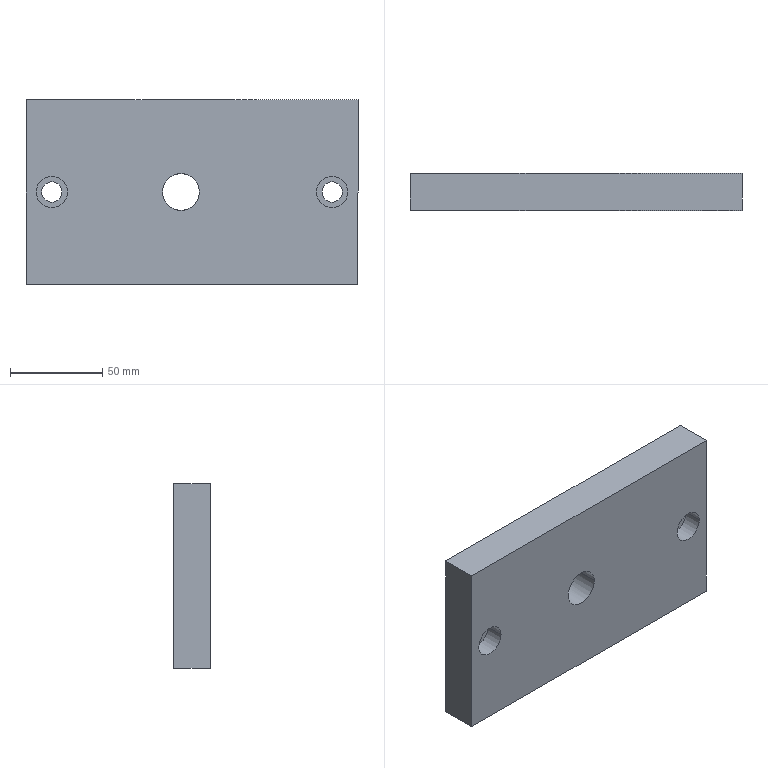Component | SolidWorks | SHYTJ-01-07-04PressurePlate-1 | 1 solid | 24 faces | box 180 x 20 x 100 mm | volume 345962 mm3 | cylinder 14 | plane 10 | commonest cylinder face diameters 20 x6 17 x4 11 x4
build123d program:
from build123d import *

# Parameters (mm, degrees)
SKETCH1_2_W             = 180
SKETCH1_2_H             = 100
BOSS_EXTRUDE1_DEPTH     = 20
SKETCH2_R               = 5
CUT_EXTRUDE1_2_DEPTH    = 207.882
SKETCH3_R               = 5.5
CUT_EXTRUDE2_DEPTH      = 207.882
SKETCH5_R               = 10
CUT_EXTRUDE3_DEPTH      = 3
SKETCH9_R               = 8.5
CUT_EXTRUDE4_DEPTH      = 10
M20X1_5_TAPPED_HOLE1_D  = 18.5
CUT_EXTRUDE1_DEPTH      = 207.882
CUT_EXTRUDE1_DEPTH_BACK = 207.882
SKETCH1_R               = 10


with BuildPart() as part:
    # Sketch1_2 → Boss-Extrude1 (new body)
    with BuildSketch(Plane.XY):
        with Locations((90, -50)):
            Rectangle(SKETCH1_2_W, SKETCH1_2_H)
    extrude(amount=BOSS_EXTRUDE1_DEPTH)

    # Sketch2 → Cut-Extrude1_2 (cut, through all)
    with BuildSketch(Plane.XY.offset(20)):
        with Locations((84, -50)):
            Circle(SKETCH2_R)
    extrude(amount=-CUT_EXTRUDE1_2_DEPTH, mode=Mode.SUBTRACT)

    # Sketch3 → Cut-Extrude2 (cut, through all)
    with BuildSketch(Plane.XY.offset(20)):
        with Locations((14, -50)):
            Circle(SKETCH3_R)
        with Locations((166, -50)):
            Circle(SKETCH3_R)
    extrude(amount=-CUT_EXTRUDE2_DEPTH, mode=Mode.SUBTRACT)

    # Sketch5 → Cut-Extrude3 (cut)
    with BuildSketch(Plane(origin=(0, 0, 0), x_dir=(-1, 0, 0), z_dir=(0, 0, -1))):
        with Locations((-14, -50)):
            Circle(SKETCH5_R)
        with Locations((-166, -50)):
            Circle(SKETCH5_R)
    extrude(amount=-CUT_EXTRUDE3_DEPTH, mode=Mode.SUBTRACT)

    # Sketch9 → Cut-Extrude4 (cut)
    with BuildSketch(Plane.XY.offset(20)):
        with Locations((14, -50)):
            Circle(SKETCH9_R)
        with Locations((166, -50)):
            Circle(SKETCH9_R)
    extrude(amount=-CUT_EXTRUDE4_DEPTH, mode=Mode.SUBTRACT)

    # M20x1.5 Tapped Hole1 (through all)
    with Locations(Plane.XY.offset(20)):
        with Locations((84, -50)):
            Hole(M20X1_5_TAPPED_HOLE1_D / 2)

    # Sketch1 → Cut-Extrude1 (cut, two sides: drawn at the far end of the back side and taken through both)
    with BuildSketch(Plane.XY.offset(-CUT_EXTRUDE1_DEPTH_BACK)):
        with Locations((84, -50)):
            Circle(SKETCH1_R)
    extrude(amount=CUT_EXTRUDE1_DEPTH + CUT_EXTRUDE1_DEPTH_BACK, mode=Mode.SUBTRACT)


solid = part.part

# Placed as in the assembly
solid = solid.moved(Location((-64.116, -45.361, 320), (90, 0, 0)))
STEP:
#1=COLOUR_RGB('',0.7922,0.8196,0.9333);
#2=FILL_AREA_STYLE_COLOUR('',#1);
#3=FILL_AREA_STYLE('',(#2));
#4=SURFACE_STYLE_FILL_AREA(#3);
#5=SURFACE_SIDE_STYLE('',(#4));
#6=SURFACE_STYLE_USAGE(.BOTH.,#5);
#7=PRESENTATION_STYLE_ASSIGNMENT((#6));
#8=CARTESIAN_POINT('',(0.3891,-1.786,10.63));
#9=VERTEX_POINT('',#8);
#10=CARTESIAN_POINT('',(1.177,-1.786,10.63));
#11=VERTEX_POINT('',#10);
#12=CARTESIAN_POINT('',(0.3891,-1.786,10.63));
#13=CARTESIAN_POINT('',(0.3891,-1.786,10.578));
#14=CARTESIAN_POINT('',(0.3991,-1.786,10.527));
#15=CARTESIAN_POINT('',(0.4391,-1.786,10.431));
#16=CARTESIAN_POINT('',(0.4675,-1.786,10.388));
#17=CARTESIAN_POINT('',(0.5414,-1.786,10.315));
#18=CARTESIAN_POINT('',(0.584,-1.786,10.286));
#19=CARTESIAN_POINT('',(0.6804,-1.786,10.246));
#20=CARTESIAN_POINT('',(0.7306,-1.786,10.236));
#21=CARTESIAN_POINT('',(0.835,-1.786,10.236));
#22=CARTESIAN_POINT('',(0.8853,-1.786,10.246));
#23=CARTESIAN_POINT('',(0.9817,-1.786,10.286));
#24=CARTESIAN_POINT('',(1.024,-1.786,10.315));
#25=CARTESIAN_POINT('',(1.098,-1.786,10.388));
#26=CARTESIAN_POINT('',(1.127,-1.786,10.431));
#27=CARTESIAN_POINT('',(1.167,-1.786,10.527));
#28=CARTESIAN_POINT('',(1.177,-1.786,10.578));
#29=CARTESIAN_POINT('',(1.177,-1.786,10.63));
#30=B_SPLINE_CURVE_WITH_KNOTS('',3,(#12,#13,#14,#15,#16,#17,#18,#19,#20,#21,#22,#23,#24,#25,#26,#27,#28,#29),.UNSPECIFIED.,.F.,.F.,(4,2,2,2,2,2,2,2,4),(0.5,0.5625,0.625,0.6875,0.75,0.8125,0.875,0.9375,1.),.UNSPECIFIED.);
#31=EDGE_CURVE('',#9,#11,#30,.T.);
#32=ORIENTED_EDGE('',*,*,#31,.F.);
#33=CARTESIAN_POINT('',(0.3891,-2.573,10.63));
#34=VERTEX_POINT('',#33);
#35=CARTESIAN_POINT('',(0.3891,-1.786,10.63));
#36=DIRECTION('',(-0.,-1.,-0.));
#37=VECTOR('',#36,39.37);
#38=LINE('',#35,#37);
#39=EDGE_CURVE('',#9,#34,#38,.T.);
#40=ORIENTED_EDGE('',*,*,#39,.T.);
#41=CARTESIAN_POINT('',(1.177,-2.573,10.63));
#42=VERTEX_POINT('',#41);
#43=CARTESIAN_POINT('',(0.7828,-2.573,10.63));
#44=DIRECTION('',(-0.,-1.,-0.));
#45=DIRECTION('',(1.,0.,0.));
#46=AXIS2_PLACEMENT_3D('',#43,#44,#45);
#47=CIRCLE('',#46,0.3937);
#48=EDGE_CURVE('',#34,#42,#47,.T.);
#49=ORIENTED_EDGE('',*,*,#48,.T.);
#50=CARTESIAN_POINT('',(1.177,-1.786,10.63));
#51=DIRECTION('',(-0.,-1.,-0.));
#52=VECTOR('',#51,39.37);
#53=LINE('',#50,#52);
#54=EDGE_CURVE('',#11,#42,#53,.T.);
#55=ORIENTED_EDGE('',*,*,#54,.F.);
#56=EDGE_LOOP('',(#32,#40,#49,#55));
#57=FACE_OUTER_BOUND('',#56,.T.);
#58=CARTESIAN_POINT('',(0.7828,-1.786,10.63));
#59=DIRECTION('',(-0.,-1.,-0.));
#60=DIRECTION('',(1.,0.,0.));
#61=AXIS2_PLACEMENT_3D('',#58,#59,#60);
#62=CYLINDRICAL_SURFACE('',#61,0.3937);
#63=ADVANCED_FACE('',(#57),#62,.F.);
#64=CARTESIAN_POINT('',(3.677,-2.18,10.63));
#65=VERTEX_POINT('',#64);
#66=CARTESIAN_POINT('',(4.346,-2.18,10.63));
#67=VERTEX_POINT('',#66);
#68=CARTESIAN_POINT('',(4.011,-2.18,10.63));
#69=DIRECTION('',(-0.,-1.,-0.));
#70=DIRECTION('',(1.,0.,0.));
#71=AXIS2_PLACEMENT_3D('',#68,#69,#70);
#72=CIRCLE('',#71,0.3346);
#73=EDGE_CURVE('',#65,#67,#72,.T.);
#74=ORIENTED_EDGE('',*,*,#73,.F.);
#75=CARTESIAN_POINT('',(3.677,-2.573,10.63));
#76=VERTEX_POINT('',#75);
#77=CARTESIAN_POINT('',(3.677,-2.18,10.63));
#78=DIRECTION('',(-0.,-1.,-0.));
#79=VECTOR('',#78,39.37);
#80=LINE('',#77,#79);
#81=EDGE_CURVE('',#65,#76,#80,.T.);
#82=ORIENTED_EDGE('',*,*,#81,.T.);
#83=CARTESIAN_POINT('',(4.346,-2.573,10.63));
#84=VERTEX_POINT('',#83);
#85=CARTESIAN_POINT('',(4.011,-2.573,10.63));
#86=DIRECTION('',(-0.,-1.,-0.));
#87=DIRECTION('',(1.,0.,0.));
#88=AXIS2_PLACEMENT_3D('',#85,#86,#87);
#89=CIRCLE('',#88,0.3346);
#90=EDGE_CURVE('',#76,#84,#89,.T.);
#91=ORIENTED_EDGE('',*,*,#90,.T.);
#92=CARTESIAN_POINT('',(4.346,-2.18,10.63));
#93=DIRECTION('',(-0.,-1.,-0.));
#94=VECTOR('',#93,39.37);
#95=LINE('',#92,#94);
#96=EDGE_CURVE('',#67,#84,#95,.T.);
#97=ORIENTED_EDGE('',*,*,#96,.F.);
#98=EDGE_LOOP('',(#74,#82,#91,#97));
#99=FACE_OUTER_BOUND('',#98,.T.);
#100=CARTESIAN_POINT('',(4.011,-2.18,10.63));
#101=DIRECTION('',(-0.,-1.,-0.));
#102=DIRECTION('',(1.,0.,0.));
#103=AXIS2_PLACEMENT_3D('',#100,#101,#102);
#104=CYLINDRICAL_SURFACE('',#103,0.3346);
#105=ADVANCED_FACE('',(#99),#104,.F.);
#106=CARTESIAN_POINT('',(-2.308,-2.18,10.63));
#107=VERTEX_POINT('',#106);
#108=CARTESIAN_POINT('',(-1.638,-2.18,10.63));
#109=VERTEX_POINT('',#108);
#110=CARTESIAN_POINT('',(-1.973,-2.18,10.63));
#111=DIRECTION('',(-0.,-1.,-0.));
#112=DIRECTION('',(1.,0.,0.));
#113=AXIS2_PLACEMENT_3D('',#110,#111,#112);
#114=CIRCLE('',#113,0.3346);
#115=EDGE_CURVE('',#107,#109,#114,.T.);
#116=ORIENTED_EDGE('',*,*,#115,.F.);
#117=CARTESIAN_POINT('',(-2.308,-2.573,10.63));
#118=VERTEX_POINT('',#117);
#119=CARTESIAN_POINT('',(-2.308,-2.18,10.63));
#120=DIRECTION('',(-0.,-1.,-0.));
#121=VECTOR('',#120,39.37);
#122=LINE('',#119,#121);
#123=EDGE_CURVE('',#107,#118,#122,.T.);
#124=ORIENTED_EDGE('',*,*,#123,.T.);
#125=CARTESIAN_POINT('',(-1.638,-2.573,10.63));
#126=VERTEX_POINT('',#125);
#127=CARTESIAN_POINT('',(-1.973,-2.573,10.63));
#128=DIRECTION('',(-0.,-1.,-0.));
#129=DIRECTION('',(1.,0.,0.));
#130=AXIS2_PLACEMENT_3D('',#127,#128,#129);
#131=CIRCLE('',#130,0.3346);
#132=EDGE_CURVE('',#118,#126,#131,.T.);
#133=ORIENTED_EDGE('',*,*,#132,.T.);
#134=CARTESIAN_POINT('',(-1.638,-2.18,10.63));
#135=DIRECTION('',(-0.,-1.,-0.));
#136=VECTOR('',#135,39.37);
#137=LINE('',#134,#136);
#138=EDGE_CURVE('',#109,#126,#137,.T.);
#139=ORIENTED_EDGE('',*,*,#138,.F.);
#140=EDGE_LOOP('',(#116,#124,#133,#139));
#141=FACE_OUTER_BOUND('',#140,.T.);
#142=CARTESIAN_POINT('',(-1.973,-2.18,10.63));
#143=DIRECTION('',(-0.,-1.,-0.));
#144=DIRECTION('',(1.,0.,0.));
#145=AXIS2_PLACEMENT_3D('',#142,#143,#144);
#146=CYLINDRICAL_SURFACE('',#145,0.3346);
#147=ADVANCED_FACE('',(#141),#146,.F.);
#148=CARTESIAN_POINT('',(4.405,-1.904,10.63));
#149=VERTEX_POINT('',#148);
#150=CARTESIAN_POINT('',(3.617,-1.904,10.63));
#151=VERTEX_POINT('',#150);
#152=CARTESIAN_POINT('',(4.011,-1.904,10.63));
#153=DIRECTION('',(0.,1.,0.));
#154=DIRECTION('',(-1.,0.,0.));
#155=AXIS2_PLACEMENT_3D('',#152,#153,#154);
#156=CIRCLE('',#155,0.3937);
#157=EDGE_CURVE('',#149,#151,#156,.T.);
#158=ORIENTED_EDGE('',*,*,#157,.F.);
#159=CARTESIAN_POINT('',(4.405,-1.786,10.63));
#160=VERTEX_POINT('',#159);
#161=CARTESIAN_POINT('',(4.405,-1.904,10.63));
#162=DIRECTION('',(0.,1.,0.));
#163=VECTOR('',#162,39.37);
#164=LINE('',#161,#163);
#165=EDGE_CURVE('',#149,#160,#164,.T.);
#166=ORIENTED_EDGE('',*,*,#165,.T.);
#167=CARTESIAN_POINT('',(3.617,-1.786,10.63));
#168=VERTEX_POINT('',#167);
#169=CARTESIAN_POINT('',(4.011,-1.786,10.63));
#170=DIRECTION('',(0.,1.,0.));
#171=DIRECTION('',(-1.,0.,0.));
#172=AXIS2_PLACEMENT_3D('',#169,#170,#171);
#173=CIRCLE('',#172,0.3937);
#174=EDGE_CURVE('',#160,#168,#173,.T.);
#175=ORIENTED_EDGE('',*,*,#174,.T.);
#176=CARTESIAN_POINT('',(3.617,-1.904,10.63));
#177=DIRECTION('',(0.,1.,0.));
#178=VECTOR('',#177,39.37);
#179=LINE('',#176,#178);
#180=EDGE_CURVE('',#151,#168,#179,.T.);
#181=ORIENTED_EDGE('',*,*,#180,.F.);
#182=EDGE_LOOP('',(#158,#166,#175,#181));
#183=FACE_OUTER_BOUND('',#182,.T.);
#184=CARTESIAN_POINT('',(4.011,-1.904,10.63));
#185=DIRECTION('',(0.,1.,0.));
#186=DIRECTION('',(-1.,0.,0.));
#187=AXIS2_PLACEMENT_3D('',#184,#185,#186);
#188=CYLINDRICAL_SURFACE('',#187,0.3937);
#189=ADVANCED_FACE('',(#183),#188,.F.);
#190=CARTESIAN_POINT('',(-1.579,-1.904,10.63));
#191=VERTEX_POINT('',#190);
#192=CARTESIAN_POINT('',(-2.367,-1.904,10.63));
#193=VERTEX_POINT('',#192);
#194=CARTESIAN_POINT('',(-1.973,-1.904,10.63));
#195=DIRECTION('',(0.,1.,0.));
#196=DIRECTION('',(-1.,0.,0.));
#197=AXIS2_PLACEMENT_3D('',#194,#195,#196);
#198=CIRCLE('',#197,0.3937);
#199=EDGE_CURVE('',#191,#193,#198,.T.);
#200=ORIENTED_EDGE('',*,*,#199,.F.);
#201=CARTESIAN_POINT('',(-1.579,-1.786,10.63));
#202=VERTEX_POINT('',#201);
#203=CARTESIAN_POINT('',(-1.579,-1.904,10.63));
#204=DIRECTION('',(0.,1.,0.));
#205=VECTOR('',#204,39.37);
#206=LINE('',#203,#205);
#207=EDGE_CURVE('',#191,#202,#206,.T.);
#208=ORIENTED_EDGE('',*,*,#207,.T.);
#209=CARTESIAN_POINT('',(-2.367,-1.786,10.63));
#210=VERTEX_POINT('',#209);
#211=CARTESIAN_POINT('',(-1.973,-1.786,10.63));
#212=DIRECTION('',(0.,1.,0.));
#213=DIRECTION('',(-1.,0.,0.));
#214=AXIS2_PLACEMENT_3D('',#211,#212,#213);
#215=CIRCLE('',#214,0.3937);
#216=EDGE_CURVE('',#202,#210,#215,.T.);
#217=ORIENTED_EDGE('',*,*,#216,.T.);
#218=CARTESIAN_POINT('',(-2.367,-1.904,10.63));
#219=DIRECTION('',(0.,1.,0.));
#220=VECTOR('',#219,39.37);
#221=LINE('',#218,#220);
#222=EDGE_CURVE('',#193,#210,#221,.T.);
#223=ORIENTED_EDGE('',*,*,#222,.F.);
#224=EDGE_LOOP('',(#200,#208,#217,#223));
#225=FACE_OUTER_BOUND('',#224,.T.);
#226=CARTESIAN_POINT('',(-1.973,-1.904,10.63));
#227=DIRECTION('',(0.,1.,0.));
#228=DIRECTION('',(-1.,0.,0.));
#229=AXIS2_PLACEMENT_3D('',#226,#227,#228);
#230=CYLINDRICAL_SURFACE('',#229,0.3937);
#231=ADVANCED_FACE('',(#225),#230,.F.);
#232=CARTESIAN_POINT('',(-2.19,-1.904,10.63));
#233=VERTEX_POINT('',#232);
#234=CARTESIAN_POINT('',(-1.757,-1.904,10.63));
#235=VERTEX_POINT('',#234);
#236=CARTESIAN_POINT('',(-1.973,-1.904,10.63));
#237=DIRECTION('',(-0.,-1.,-0.));
#238=DIRECTION('',(-1.,0.,0.));
#239=AXIS2_PLACEMENT_3D('',#236,#237,#238);
#240=CIRCLE('',#239,0.2165);
#241=EDGE_CURVE('',#233,#235,#240,.T.);
#242=ORIENTED_EDGE('',*,*,#241,.F.);
#243=CARTESIAN_POINT('',(-2.19,-2.18,10.63));
#244=VERTEX_POINT('',#243);
#245=CARTESIAN_POINT('',(-2.19,-1.786,10.63));
#246=DIRECTION('',(-0.,-1.,-0.));
#247=VECTOR('',#246,39.37);
#248=LINE('',#245,#247);
#249=EDGE_CURVE('',#233,#244,#248,.T.);
#250=ORIENTED_EDGE('',*,*,#249,.T.);
#251=CARTESIAN_POINT('',(-1.757,-2.18,10.63));
#252=VERTEX_POINT('',#251);
#253=CARTESIAN_POINT('',(-1.973,-2.18,10.63));
#254=DIRECTION('',(0.,1.,0.));
#255=DIRECTION('',(1.,0.,0.));
#256=AXIS2_PLACEMENT_3D('',#253,#254,#255);
#257=CIRCLE('',#256,0.2165);
#258=EDGE_CURVE('',#252,#244,#257,.T.);
#259=ORIENTED_EDGE('',*,*,#258,.F.);
#260=CARTESIAN_POINT('',(-1.757,-1.786,10.63));
#261=DIRECTION('',(-0.,-1.,-0.));
#262=VECTOR('',#261,39.37);
#263=LINE('',#260,#262);
#264=EDGE_CURVE('',#235,#252,#263,.T.);
#265=ORIENTED_EDGE('',*,*,#264,.F.);
#266=EDGE_LOOP('',(#242,#250,#259,#265));
#267=FACE_OUTER_BOUND('',#266,.T.);
#268=CARTESIAN_POINT('',(-1.973,-1.786,10.63));
#269=DIRECTION('',(-0.,-1.,-0.));
#270=DIRECTION('',(1.,0.,0.));
#271=AXIS2_PLACEMENT_3D('',#268,#269,#270);
#272=CYLINDRICAL_SURFACE('',#271,0.2165);
#273=ADVANCED_FACE('',(#267),#272,.F.);
#274=CARTESIAN_POINT('',(3.795,-1.904,10.63));
#275=VERTEX_POINT('',#274);
#276=CARTESIAN_POINT('',(4.228,-1.904,10.63));
#277=VERTEX_POINT('',#276);
#278=CARTESIAN_POINT('',(4.011,-1.904,10.63));
#279=DIRECTION('',(-0.,-1.,-0.));
#280=DIRECTION('',(-1.,0.,0.));
#281=AXIS2_PLACEMENT_3D('',#278,#279,#280);
#282=CIRCLE('',#281,0.2165);
#283=EDGE_CURVE('',#275,#277,#282,.T.);
#284=ORIENTED_EDGE('',*,*,#283,.F.);
#285=CARTESIAN_POINT('',(3.795,-2.18,10.63));
#286=VERTEX_POINT('',#285);
#287=CARTESIAN_POINT('',(3.795,-1.786,10.63));
#288=DIRECTION('',(-0.,-1.,-0.));
#289=VECTOR('',#288,39.37);
#290=LINE('',#287,#289);
#291=EDGE_CURVE('',#275,#286,#290,.T.);
#292=ORIENTED_EDGE('',*,*,#291,.T.);
#293=CARTESIAN_POINT('',(4.228,-2.18,10.63));
#294=VERTEX_POINT('',#293);
#295=CARTESIAN_POINT('',(4.011,-2.18,10.63));
#296=DIRECTION('',(0.,1.,0.));
#297=DIRECTION('',(1.,0.,0.));
#298=AXIS2_PLACEMENT_3D('',#295,#296,#297);
#299=CIRCLE('',#298,0.2165);
#300=EDGE_CURVE('',#294,#286,#299,.T.);
#301=ORIENTED_EDGE('',*,*,#300,.F.);
#302=CARTESIAN_POINT('',(4.228,-1.786,10.63));
#303=DIRECTION('',(-0.,-1.,-0.));
#304=VECTOR('',#303,39.37);
#305=LINE('',#302,#304);
#306=EDGE_CURVE('',#277,#294,#305,.T.);
#307=ORIENTED_EDGE('',*,*,#306,.F.);
#308=EDGE_LOOP('',(#284,#292,#301,#307));
#309=FACE_OUTER_BOUND('',#308,.T.);
#310=CARTESIAN_POINT('',(4.011,-1.786,10.63));
#311=DIRECTION('',(-0.,-1.,-0.));
#312=DIRECTION('',(1.,0.,0.));
#313=AXIS2_PLACEMENT_3D('',#310,#311,#312);
#314=CYLINDRICAL_SURFACE('',#313,0.2165);
#315=ADVANCED_FACE('',(#309),#314,.F.);
#316=ORIENTED_EDGE('',*,*,#291,.F.);
#317=CARTESIAN_POINT('',(4.011,-1.904,10.63));
#318=DIRECTION('',(-0.,-1.,-0.));
#319=DIRECTION('',(-1.,0.,0.));
#320=AXIS2_PLACEMENT_3D('',#317,#318,#319);
#321=CIRCLE('',#320,0.2165);
#322=EDGE_CURVE('',#277,#275,#321,.T.);
#323=ORIENTED_EDGE('',*,*,#322,.F.);
#324=ORIENTED_EDGE('',*,*,#306,.T.);
#325=CARTESIAN_POINT('',(4.011,-2.18,10.63));
#326=DIRECTION('',(0.,1.,0.));
#327=DIRECTION('',(1.,0.,0.));
#328=AXIS2_PLACEMENT_3D('',#325,#326,#327);
#329=CIRCLE('',#328,0.2165);
#330=EDGE_CURVE('',#286,#294,#329,.T.);
#331=ORIENTED_EDGE('',*,*,#330,.F.);
#332=EDGE_LOOP('',(#316,#323,#324,#331));
#333=FACE_OUTER_BOUND('',#332,.T.);
#334=CARTESIAN_POINT('',(4.011,-1.786,10.63));
#335=DIRECTION('',(-0.,-1.,-0.));
#336=DIRECTION('',(1.,0.,0.));
#337=AXIS2_PLACEMENT_3D('',#334,#335,#336);
#338=CYLINDRICAL_SURFACE('',#337,0.2165);
#339=ADVANCED_FACE('',(#333),#338,.F.);
#340=ORIENTED_EDGE('',*,*,#249,.F.);
#341=CARTESIAN_POINT('',(-1.973,-1.904,10.63));
#342=DIRECTION('',(-0.,-1.,-0.));
#343=DIRECTION('',(-1.,0.,0.));
#344=AXIS2_PLACEMENT_3D('',#341,#342,#343);
#345=CIRCLE('',#344,0.2165);
#346=EDGE_CURVE('',#235,#233,#345,.T.);
#347=ORIENTED_EDGE('',*,*,#346,.F.);
#348=ORIENTED_EDGE('',*,*,#264,.T.);
#349=CARTESIAN_POINT('',(-1.973,-2.18,10.63));
#350=DIRECTION('',(0.,1.,0.));
#351=DIRECTION('',(1.,0.,0.));
#352=AXIS2_PLACEMENT_3D('',#349,#350,#351);
#353=CIRCLE('',#352,0.2165);
#354=EDGE_CURVE('',#244,#252,#353,.T.);
#355=ORIENTED_EDGE('',*,*,#354,.F.);
#356=EDGE_LOOP('',(#340,#347,#348,#355));
#357=FACE_OUTER_BOUND('',#356,.T.);
#358=CARTESIAN_POINT('',(-1.973,-1.786,10.63));
#359=DIRECTION('',(-0.,-1.,-0.));
#360=DIRECTION('',(1.,0.,0.));
#361=AXIS2_PLACEMENT_3D('',#358,#359,#360);
#362=CYLINDRICAL_SURFACE('',#361,0.2165);
#363=ADVANCED_FACE('',(#357),#362,.F.);
#364=CARTESIAN_POINT('',(-2.524,-1.786,12.598));
#365=VERTEX_POINT('',#364);
#366=CARTESIAN_POINT('',(-2.524,-1.786,8.661));
#367=VERTEX_POINT('',#366);
#368=CARTESIAN_POINT('',(-2.524,-1.786,12.598));
#369=DIRECTION('',(-0.,0.,-1.));
#370=VECTOR('',#369,39.37);
#371=LINE('',#368,#370);
#372=EDGE_CURVE('',#365,#367,#371,.T.);
#373=ORIENTED_EDGE('',*,*,#372,.T.);
#374=CARTESIAN_POINT('',(-2.524,-2.573,8.661));
#375=VERTEX_POINT('',#374);
#376=CARTESIAN_POINT('',(-2.524,-2.573,8.661));
#377=DIRECTION('',(0.,1.,0.));
#378=VECTOR('',#377,39.37);
#379=LINE('',#376,#378);
#380=EDGE_CURVE('',#375,#367,#379,.T.);
#381=ORIENTED_EDGE('',*,*,#380,.F.);
#382=CARTESIAN_POINT('',(-2.524,-2.573,12.598));
#383=VERTEX_POINT('',#382);
#384=CARTESIAN_POINT('',(-2.524,-2.573,12.598));
#385=DIRECTION('',(-0.,0.,-1.));
#386=VECTOR('',#385,39.37);
#387=LINE('',#384,#386);
#388=EDGE_CURVE('',#383,#375,#387,.T.);
#389=ORIENTED_EDGE('',*,*,#388,.F.);
#390=CARTESIAN_POINT('',(-2.524,-2.573,12.598));
#391=DIRECTION('',(0.,1.,0.));
#392=VECTOR('',#391,39.37);
#393=LINE('',#390,#392);
#394=EDGE_CURVE('',#383,#365,#393,.T.);
#395=ORIENTED_EDGE('',*,*,#394,.T.);
#396=EDGE_LOOP('',(#373,#381,#389,#395));
#397=FACE_OUTER_BOUND('',#396,.T.);
#398=CARTESIAN_POINT('',(-2.524,-2.573,12.598));
#399=DIRECTION('',(1.,-0.,-0.));
#400=DIRECTION('',(0.,-0.,1.));
#401=AXIS2_PLACEMENT_3D('',#398,#399,#400);
#402=PLANE('',#401);
#403=ADVANCED_FACE('',(#397),#402,.F.);
#404=CARTESIAN_POINT('',(4.562,-1.786,8.661));
#405=VERTEX_POINT('',#404);
#406=CARTESIAN_POINT('',(-2.524,-1.786,8.661));
#407=DIRECTION('',(1.,-0.,-0.));
#408=VECTOR('',#407,39.37);
#409=LINE('',#406,#408);
#410=EDGE_CURVE('',#367,#405,#409,.T.);
#411=ORIENTED_EDGE('',*,*,#410,.T.);
#412=CARTESIAN_POINT('',(4.562,-2.573,8.661));
#413=VERTEX_POINT('',#412);
#414=CARTESIAN_POINT('',(4.562,-2.573,8.661));
#415=DIRECTION('',(0.,1.,0.));
#416=VECTOR('',#415,39.37);
#417=LINE('',#414,#416);
#418=EDGE_CURVE('',#413,#405,#417,.T.);
#419=ORIENTED_EDGE('',*,*,#418,.F.);
#420=CARTESIAN_POINT('',(-2.524,-2.573,8.661));
#421=DIRECTION('',(1.,-0.,-0.));
#422=VECTOR('',#421,39.37);
#423=LINE('',#420,#422);
#424=EDGE_CURVE('',#375,#413,#423,.T.);
#425=ORIENTED_EDGE('',*,*,#424,.F.);
#426=ORIENTED_EDGE('',*,*,#380,.T.);
#427=EDGE_LOOP('',(#411,#419,#425,#426));
#428=FACE_OUTER_BOUND('',#427,.T.);
#429=CARTESIAN_POINT('',(-2.524,-2.573,8.661));
#430=DIRECTION('',(0.,-0.,1.));
#431=DIRECTION('',(-0.,-1.,-0.));
#432=AXIS2_PLACEMENT_3D('',#429,#430,#431);
#433=PLANE('',#432);
#434=ADVANCED_FACE('',(#428),#433,.F.);
#435=CARTESIAN_POINT('',(4.562,-1.786,12.598));
#436=VERTEX_POINT('',#435);
#437=CARTESIAN_POINT('',(4.562,-1.786,12.598));
#438=DIRECTION('',(0.,-0.,1.));
#439=VECTOR('',#438,39.37);
#440=LINE('',#437,#439);
#441=EDGE_CURVE('',#405,#436,#440,.T.);
#442=ORIENTED_EDGE('',*,*,#441,.T.);
#443=CARTESIAN_POINT('',(4.562,-2.573,12.598));
#444=VERTEX_POINT('',#443);
#445=CARTESIAN_POINT('',(4.562,-2.573,12.598));
#446=DIRECTION('',(0.,1.,0.));
#447=VECTOR('',#446,39.37);
#448=LINE('',#445,#447);
#449=EDGE_CURVE('',#444,#436,#448,.T.);
#450=ORIENTED_EDGE('',*,*,#449,.F.);
#451=CARTESIAN_POINT('',(4.562,-2.573,12.598));
#452=DIRECTION('',(0.,-0.,1.));
#453=VECTOR('',#452,39.37);
#454=LINE('',#451,#453);
#455=EDGE_CURVE('',#413,#444,#454,.T.);
#456=ORIENTED_EDGE('',*,*,#455,.F.);
#457=ORIENTED_EDGE('',*,*,#418,.T.);
#458=EDGE_LOOP('',(#442,#450,#456,#457));
#459=FACE_OUTER_BOUND('',#458,.T.);
#460=CARTESIAN_POINT('',(4.562,-2.573,12.598));
#461=DIRECTION('',(-1.,0.,0.));
#462=DIRECTION('',(-0.,-1.,-0.));
#463=AXIS2_PLACEMENT_3D('',#460,#461,#462);
#464=PLANE('',#463);
#465=ADVANCED_FACE('',(#459),#464,.F.);
#466=CARTESIAN_POINT('',(-2.524,-1.786,12.598));
#467=DIRECTION('',(-1.,0.,0.));
#468=VECTOR('',#467,39.37);
#469=LINE('',#466,#468);
#470=EDGE_CURVE('',#436,#365,#469,.T.);
#471=ORIENTED_EDGE('',*,*,#470,.T.);
#472=ORIENTED_EDGE('',*,*,#394,.F.);
#473=CARTESIAN_POINT('',(-2.524,-2.573,12.598));
#474=DIRECTION('',(-1.,0.,0.));
#475=VECTOR('',#474,39.37);
#476=LINE('',#473,#475);
#477=EDGE_CURVE('',#444,#383,#476,.T.);
#478=ORIENTED_EDGE('',*,*,#477,.F.);
#479=ORIENTED_EDGE('',*,*,#449,.T.);
#480=EDGE_LOOP('',(#471,#472,#478,#479));
#481=FACE_OUTER_BOUND('',#480,.T.);
#482=CARTESIAN_POINT('',(-2.524,-2.573,12.598));
#483=DIRECTION('',(-0.,0.,-1.));
#484=DIRECTION('',(0.,1.,0.));
#485=AXIS2_PLACEMENT_3D('',#482,#483,#484);
#486=PLANE('',#485);
#487=ADVANCED_FACE('',(#481),#486,.F.);
#488=CARTESIAN_POINT('',(0.7828,-2.573,10.63));
#489=DIRECTION('',(-0.,-1.,-0.));
#490=DIRECTION('',(1.,0.,0.));
#491=AXIS2_PLACEMENT_3D('',#488,#489,#490);
#492=CIRCLE('',#491,0.3937);
#493=EDGE_CURVE('',#42,#34,#492,.T.);
#494=ORIENTED_EDGE('',*,*,#493,.F.);
#495=ORIENTED_EDGE('',*,*,#48,.F.);
#496=EDGE_LOOP('',(#494,#495));
#497=FACE_BOUND('',#496,.T.);
#498=CARTESIAN_POINT('',(4.011,-2.573,10.63));
#499=DIRECTION('',(-0.,-1.,-0.));
#500=DIRECTION('',(1.,0.,0.));
#501=AXIS2_PLACEMENT_3D('',#498,#499,#500);
#502=CIRCLE('',#501,0.3346);
#503=EDGE_CURVE('',#84,#76,#502,.T.);
#504=ORIENTED_EDGE('',*,*,#503,.F.);
#505=ORIENTED_EDGE('',*,*,#90,.F.);
#506=EDGE_LOOP('',(#504,#505));
#507=FACE_BOUND('',#506,.T.);
#508=CARTESIAN_POINT('',(-1.973,-2.573,10.63));
#509=DIRECTION('',(-0.,-1.,-0.));
#510=DIRECTION('',(1.,0.,0.));
#511=AXIS2_PLACEMENT_3D('',#508,#509,#510);
#512=CIRCLE('',#511,0.3346);
#513=EDGE_CURVE('',#126,#118,#512,.T.);
#514=ORIENTED_EDGE('',*,*,#513,.F.);
#515=ORIENTED_EDGE('',*,*,#132,.F.);
#516=EDGE_LOOP('',(#514,#515));
#517=FACE_BOUND('',#516,.T.);
#518=ORIENTED_EDGE('',*,*,#388,.T.);
#519=ORIENTED_EDGE('',*,*,#424,.T.);
#520=ORIENTED_EDGE('',*,*,#455,.T.);
#521=ORIENTED_EDGE('',*,*,#477,.T.);
#522=EDGE_LOOP('',(#518,#519,#520,#521));
#523=FACE_OUTER_BOUND('',#522,.T.);
#524=CARTESIAN_POINT('',(-2.524,-2.573,12.598));
#525=DIRECTION('',(-0.,-1.,-0.));
#526=DIRECTION('',(1.,-0.,-0.));
#527=AXIS2_PLACEMENT_3D('',#524,#525,#526);
#528=PLANE('',#527);
#529=ADVANCED_FACE('',(#497,#507,#517,#523),#528,.T.);
#530=CARTESIAN_POINT('',(1.177,-1.786,10.63));
#531=CARTESIAN_POINT('',(1.177,-1.786,10.682));
#532=CARTESIAN_POINT('',(1.167,-1.786,10.732));
#533=CARTESIAN_POINT('',(1.127,-1.786,10.829));
#534=CARTESIAN_POINT('',(1.098,-1.786,10.871));
#535=CARTESIAN_POINT('',(1.024,-1.786,10.945));
#536=CARTESIAN_POINT('',(0.9817,-1.786,10.974));
#537=CARTESIAN_POINT('',(0.8853,-1.786,11.014));
#538=CARTESIAN_POINT('',(0.835,-1.786,11.024));
#539=CARTESIAN_POINT('',(0.7306,-1.786,11.024));
#540=CARTESIAN_POINT('',(0.6804,-1.786,11.014));
#541=CARTESIAN_POINT('',(0.584,-1.786,10.974));
#542=CARTESIAN_POINT('',(0.5414,-1.786,10.945));
#543=CARTESIAN_POINT('',(0.4675,-1.786,10.871));
#544=CARTESIAN_POINT('',(0.4391,-1.786,10.829));
#545=CARTESIAN_POINT('',(0.3991,-1.786,10.732));
#546=CARTESIAN_POINT('',(0.3891,-1.786,10.682));
#547=CARTESIAN_POINT('',(0.3891,-1.786,10.63));
#548=B_SPLINE_CURVE_WITH_KNOTS('',3,(#530,#531,#532,#533,#534,#535,#536,#537,#538,#539,#540,#541,#542,#543,#544,#545,#546,#547),.UNSPECIFIED.,.F.,.F.,(4,2,2,2,2,2,2,2,4),(0.,0.0625,0.125,0.1875,0.25,0.3125,0.375,0.4375,0.5),.UNSPECIFIED.);
#549=EDGE_CURVE('',#11,#9,#548,.T.);
#550=ORIENTED_EDGE('',*,*,#549,.T.);
#551=ORIENTED_EDGE('',*,*,#31,.T.);
#552=EDGE_LOOP('',(#550,#551));
#553=FACE_BOUND('',#552,.T.);
#554=CARTESIAN_POINT('',(4.011,-1.786,10.63));
#555=DIRECTION('',(0.,1.,0.));
#556=DIRECTION('',(-1.,0.,0.));
#557=AXIS2_PLACEMENT_3D('',#554,#555,#556);
#558=CIRCLE('',#557,0.3937);
#559=EDGE_CURVE('',#168,#160,#558,.T.);
#560=ORIENTED_EDGE('',*,*,#559,.F.);
#561=ORIENTED_EDGE('',*,*,#174,.F.);
#562=EDGE_LOOP('',(#560,#561));
#563=FACE_BOUND('',#562,.T.);
#564=CARTESIAN_POINT('',(-1.973,-1.786,10.63));
#565=DIRECTION('',(0.,1.,0.));
#566=DIRECTION('',(-1.,0.,0.));
#567=AXIS2_PLACEMENT_3D('',#564,#565,#566);
#568=CIRCLE('',#567,0.3937);
#569=EDGE_CURVE('',#210,#202,#568,.T.);
#570=ORIENTED_EDGE('',*,*,#569,.F.);
#571=ORIENTED_EDGE('',*,*,#216,.F.);
#572=EDGE_LOOP('',(#570,#571));
#573=FACE_BOUND('',#572,.T.);
#574=ORIENTED_EDGE('',*,*,#372,.F.);
#575=ORIENTED_EDGE('',*,*,#470,.F.);
#576=ORIENTED_EDGE('',*,*,#441,.F.);
#577=ORIENTED_EDGE('',*,*,#410,.F.);
#578=EDGE_LOOP('',(#574,#575,#576,#577));
#579=FACE_OUTER_BOUND('',#578,.T.);
#580=CARTESIAN_POINT('',(-2.524,-1.786,12.598));
#581=DIRECTION('',(-0.,-1.,-0.));
#582=DIRECTION('',(1.,-0.,-0.));
#583=AXIS2_PLACEMENT_3D('',#580,#581,#582);
#584=PLANE('',#583);
#585=ADVANCED_FACE('',(#553,#563,#573,#579),#584,.F.);
#586=CARTESIAN_POINT('',(-1.973,-1.904,10.63));
#587=DIRECTION('',(0.,1.,0.));
#588=DIRECTION('',(-1.,0.,0.));
#589=AXIS2_PLACEMENT_3D('',#586,#587,#588);
#590=CIRCLE('',#589,0.3937);
#591=EDGE_CURVE('',#193,#191,#590,.T.);
#592=ORIENTED_EDGE('',*,*,#591,.T.);
#593=ORIENTED_EDGE('',*,*,#199,.T.);
#594=EDGE_LOOP('',(#592,#593));
#595=FACE_OUTER_BOUND('',#594,.T.);
#596=ORIENTED_EDGE('',*,*,#346,.T.);
#597=ORIENTED_EDGE('',*,*,#241,.T.);
#598=EDGE_LOOP('',(#596,#597));
#599=FACE_BOUND('',#598,.T.);
#600=CARTESIAN_POINT('',(-1.973,-1.904,10.63));
#601=DIRECTION('',(0.,1.,0.));
#602=DIRECTION('',(-1.,0.,0.));
#603=AXIS2_PLACEMENT_3D('',#600,#601,#602);
#604=PLANE('',#603);
#605=ADVANCED_FACE('',(#595,#599),#604,.T.);
#606=ORIENTED_EDGE('',*,*,#207,.F.);
#607=ORIENTED_EDGE('',*,*,#591,.F.);
#608=ORIENTED_EDGE('',*,*,#222,.T.);
#609=ORIENTED_EDGE('',*,*,#569,.T.);
#610=EDGE_LOOP('',(#606,#607,#608,#609));
#611=FACE_OUTER_BOUND('',#610,.T.);
#612=CARTESIAN_POINT('',(-1.973,-1.904,10.63));
#613=DIRECTION('',(0.,1.,0.));
#614=DIRECTION('',(-1.,0.,0.));
#615=AXIS2_PLACEMENT_3D('',#612,#613,#614);
#616=CYLINDRICAL_SURFACE('',#615,0.3937);
#617=ADVANCED_FACE('',(#611),#616,.F.);
#618=CARTESIAN_POINT('',(4.011,-1.904,10.63));
#619=DIRECTION('',(0.,1.,0.));
#620=DIRECTION('',(-1.,0.,0.));
#621=AXIS2_PLACEMENT_3D('',#618,#619,#620);
#622=CIRCLE('',#621,0.3937);
#623=EDGE_CURVE('',#151,#149,#622,.T.);
#624=ORIENTED_EDGE('',*,*,#623,.T.);
#625=ORIENTED_EDGE('',*,*,#157,.T.);
#626=EDGE_LOOP('',(#624,#625));
#627=FACE_OUTER_BOUND('',#626,.T.);
#628=ORIENTED_EDGE('',*,*,#322,.T.);
#629=ORIENTED_EDGE('',*,*,#283,.T.);
#630=EDGE_LOOP('',(#628,#629));
#631=FACE_BOUND('',#630,.T.);
#632=CARTESIAN_POINT('',(4.011,-1.904,10.63));
#633=DIRECTION('',(0.,1.,0.));
#634=DIRECTION('',(-1.,0.,0.));
#635=AXIS2_PLACEMENT_3D('',#632,#633,#634);
#636=PLANE('',#635);
#637=ADVANCED_FACE('',(#627,#631),#636,.T.);
#638=ORIENTED_EDGE('',*,*,#165,.F.);
#639=ORIENTED_EDGE('',*,*,#623,.F.);
#640=ORIENTED_EDGE('',*,*,#180,.T.);
#641=ORIENTED_EDGE('',*,*,#559,.T.);
#642=EDGE_LOOP('',(#638,#639,#640,#641));
#643=FACE_OUTER_BOUND('',#642,.T.);
#644=CARTESIAN_POINT('',(4.011,-1.904,10.63));
#645=DIRECTION('',(0.,1.,0.));
#646=DIRECTION('',(-1.,0.,0.));
#647=AXIS2_PLACEMENT_3D('',#644,#645,#646);
#648=CYLINDRICAL_SURFACE('',#647,0.3937);
#649=ADVANCED_FACE('',(#643),#648,.F.);
#650=CARTESIAN_POINT('',(-1.973,-2.18,10.63));
#651=DIRECTION('',(-0.,-1.,-0.));
#652=DIRECTION('',(1.,0.,0.));
#653=AXIS2_PLACEMENT_3D('',#650,#651,#652);
#654=CIRCLE('',#653,0.3346);
#655=EDGE_CURVE('',#109,#107,#654,.T.);
#656=ORIENTED_EDGE('',*,*,#655,.T.);
#657=ORIENTED_EDGE('',*,*,#115,.T.);
#658=EDGE_LOOP('',(#656,#657));
#659=FACE_OUTER_BOUND('',#658,.T.);
#660=ORIENTED_EDGE('',*,*,#258,.T.);
#661=ORIENTED_EDGE('',*,*,#354,.T.);
#662=EDGE_LOOP('',(#660,#661));
#663=FACE_BOUND('',#662,.T.);
#664=CARTESIAN_POINT('',(-1.973,-2.18,10.63));
#665=DIRECTION('',(-0.,-1.,-0.));
#666=DIRECTION('',(1.,-0.,-0.));
#667=AXIS2_PLACEMENT_3D('',#664,#665,#666);
#668=PLANE('',#667);
#669=ADVANCED_FACE('',(#659,#663),#668,.T.);
#670=ORIENTED_EDGE('',*,*,#123,.F.);
#671=ORIENTED_EDGE('',*,*,#655,.F.);
#672=ORIENTED_EDGE('',*,*,#138,.T.);
#673=ORIENTED_EDGE('',*,*,#513,.T.);
#674=EDGE_LOOP('',(#670,#671,#672,#673));
#675=FACE_OUTER_BOUND('',#674,.T.);
#676=CARTESIAN_POINT('',(-1.973,-2.18,10.63));
#677=DIRECTION('',(-0.,-1.,-0.));
#678=DIRECTION('',(1.,0.,0.));
#679=AXIS2_PLACEMENT_3D('',#676,#677,#678);
#680=CYLINDRICAL_SURFACE('',#679,0.3346);
#681=ADVANCED_FACE('',(#675),#680,.F.);
#682=CARTESIAN_POINT('',(4.011,-2.18,10.63));
#683=DIRECTION('',(-0.,-1.,-0.));
#684=DIRECTION('',(1.,0.,0.));
#685=AXIS2_PLACEMENT_3D('',#682,#683,#684);
#686=CIRCLE('',#685,0.3346);
#687=EDGE_CURVE('',#67,#65,#686,.T.);
#688=ORIENTED_EDGE('',*,*,#687,.T.);
#689=ORIENTED_EDGE('',*,*,#73,.T.);
#690=EDGE_LOOP('',(#688,#689));
#691=FACE_OUTER_BOUND('',#690,.T.);
#692=ORIENTED_EDGE('',*,*,#300,.T.);
#693=ORIENTED_EDGE('',*,*,#330,.T.);
#694=EDGE_LOOP('',(#692,#693));
#695=FACE_BOUND('',#694,.T.);
#696=CARTESIAN_POINT('',(4.011,-2.18,10.63));
#697=DIRECTION('',(-0.,-1.,-0.));
#698=DIRECTION('',(1.,-0.,-0.));
#699=AXIS2_PLACEMENT_3D('',#696,#697,#698);
#700=PLANE('',#699);
#701=ADVANCED_FACE('',(#691,#695),#700,.T.);
#702=ORIENTED_EDGE('',*,*,#81,.F.);
#703=ORIENTED_EDGE('',*,*,#687,.F.);
#704=ORIENTED_EDGE('',*,*,#96,.T.);
#705=ORIENTED_EDGE('',*,*,#503,.T.);
#706=EDGE_LOOP('',(#702,#703,#704,#705));
#707=FACE_OUTER_BOUND('',#706,.T.);
#708=CARTESIAN_POINT('',(4.011,-2.18,10.63));
#709=DIRECTION('',(-0.,-1.,-0.));
#710=DIRECTION('',(1.,0.,0.));
#711=AXIS2_PLACEMENT_3D('',#708,#709,#710);
#712=CYLINDRICAL_SURFACE('',#711,0.3346);
#713=ADVANCED_FACE('',(#707),#712,.F.);
#714=ORIENTED_EDGE('',*,*,#39,.F.);
#715=ORIENTED_EDGE('',*,*,#549,.F.);
#716=ORIENTED_EDGE('',*,*,#54,.T.);
#717=ORIENTED_EDGE('',*,*,#493,.T.);
#718=EDGE_LOOP('',(#714,#715,#716,#717));
#719=FACE_OUTER_BOUND('',#718,.T.);
#720=CARTESIAN_POINT('',(0.7828,-1.786,10.63));
#721=DIRECTION('',(-0.,-1.,-0.));
#722=DIRECTION('',(1.,0.,0.));
#723=AXIS2_PLACEMENT_3D('',#720,#721,#722);
#724=CYLINDRICAL_SURFACE('',#723,0.3937);
#725=ADVANCED_FACE('',(#719),#724,.F.);
#726=CLOSED_SHELL('',(#63,#105,#147,#189,#231,#273,#315,#339,#363,#403,#434,#465,#487,#529,#585,#605,#617,#637,#649,#669,#681,#701,#713,#725));
#727=MANIFOLD_SOLID_BREP('',#726);
#728=STYLED_ITEM('',(#7),#727);
#729=PRESENTATION_LAYER_ASSIGNMENT('','',(#728));
#730=(LENGTH_UNIT()NAMED_UNIT(*)SI_UNIT($,.METRE.));
#731=LENGTH_MEASURE_WITH_UNIT(LENGTH_MEASURE(0.0254),#730);
#732=DIMENSIONAL_EXPONENTS(1.,0.,0.,0.,0.,0.,0.);
#733=(CONVERSION_BASED_UNIT('',#731)LENGTH_UNIT()NAMED_UNIT(#732));
#734=UNCERTAINTY_MEASURE_WITH_UNIT(LENGTH_MEASURE(0.00001),#733,'','');
#735=(NAMED_UNIT(*)PLANE_ANGLE_UNIT()SI_UNIT($,.RADIAN.));
#736=(NAMED_UNIT(*)SI_UNIT($,.STERADIAN.)SOLID_ANGLE_UNIT());
#737=(GEOMETRIC_REPRESENTATION_CONTEXT(3)GLOBAL_UNCERTAINTY_ASSIGNED_CONTEXT((#734))GLOBAL_UNIT_ASSIGNED_CONTEXT((#733,#735,#736))REPRESENTATION_CONTEXT('',''));
#738=MECHANICAL_DESIGN_GEOMETRIC_PRESENTATION_REPRESENTATION('',(#728),#737);
#739=CARTESIAN_POINT('',(0.,0.,0.));
#740=DIRECTION('',(0.,0.,1.));
#741=DIRECTION('',(1.,0.,0.));
#742=AXIS2_PLACEMENT_3D('',#739,#740,#741);
#743=(LENGTH_UNIT()NAMED_UNIT(*)SI_UNIT($,.METRE.));
#744=LENGTH_MEASURE_WITH_UNIT(LENGTH_MEASURE(0.0254),#743);
#745=DIMENSIONAL_EXPONENTS(1.,0.,0.,0.,0.,0.,0.);
#746=(CONVERSION_BASED_UNIT('',#744)LENGTH_UNIT()NAMED_UNIT(#745));
#747=UNCERTAINTY_MEASURE_WITH_UNIT(LENGTH_MEASURE(0.00001),#746,'','');
#748=(NAMED_UNIT(*)PLANE_ANGLE_UNIT()SI_UNIT($,.RADIAN.));
#749=(NAMED_UNIT(*)SI_UNIT($,.STERADIAN.)SOLID_ANGLE_UNIT());
#750=(GEOMETRIC_REPRESENTATION_CONTEXT(3)GLOBAL_UNCERTAINTY_ASSIGNED_CONTEXT((#747))GLOBAL_UNIT_ASSIGNED_CONTEXT((#746,#748,#749))REPRESENTATION_CONTEXT('',''));
#751=ADVANCED_BREP_SHAPE_REPRESENTATION('',(#727,#742),#750);